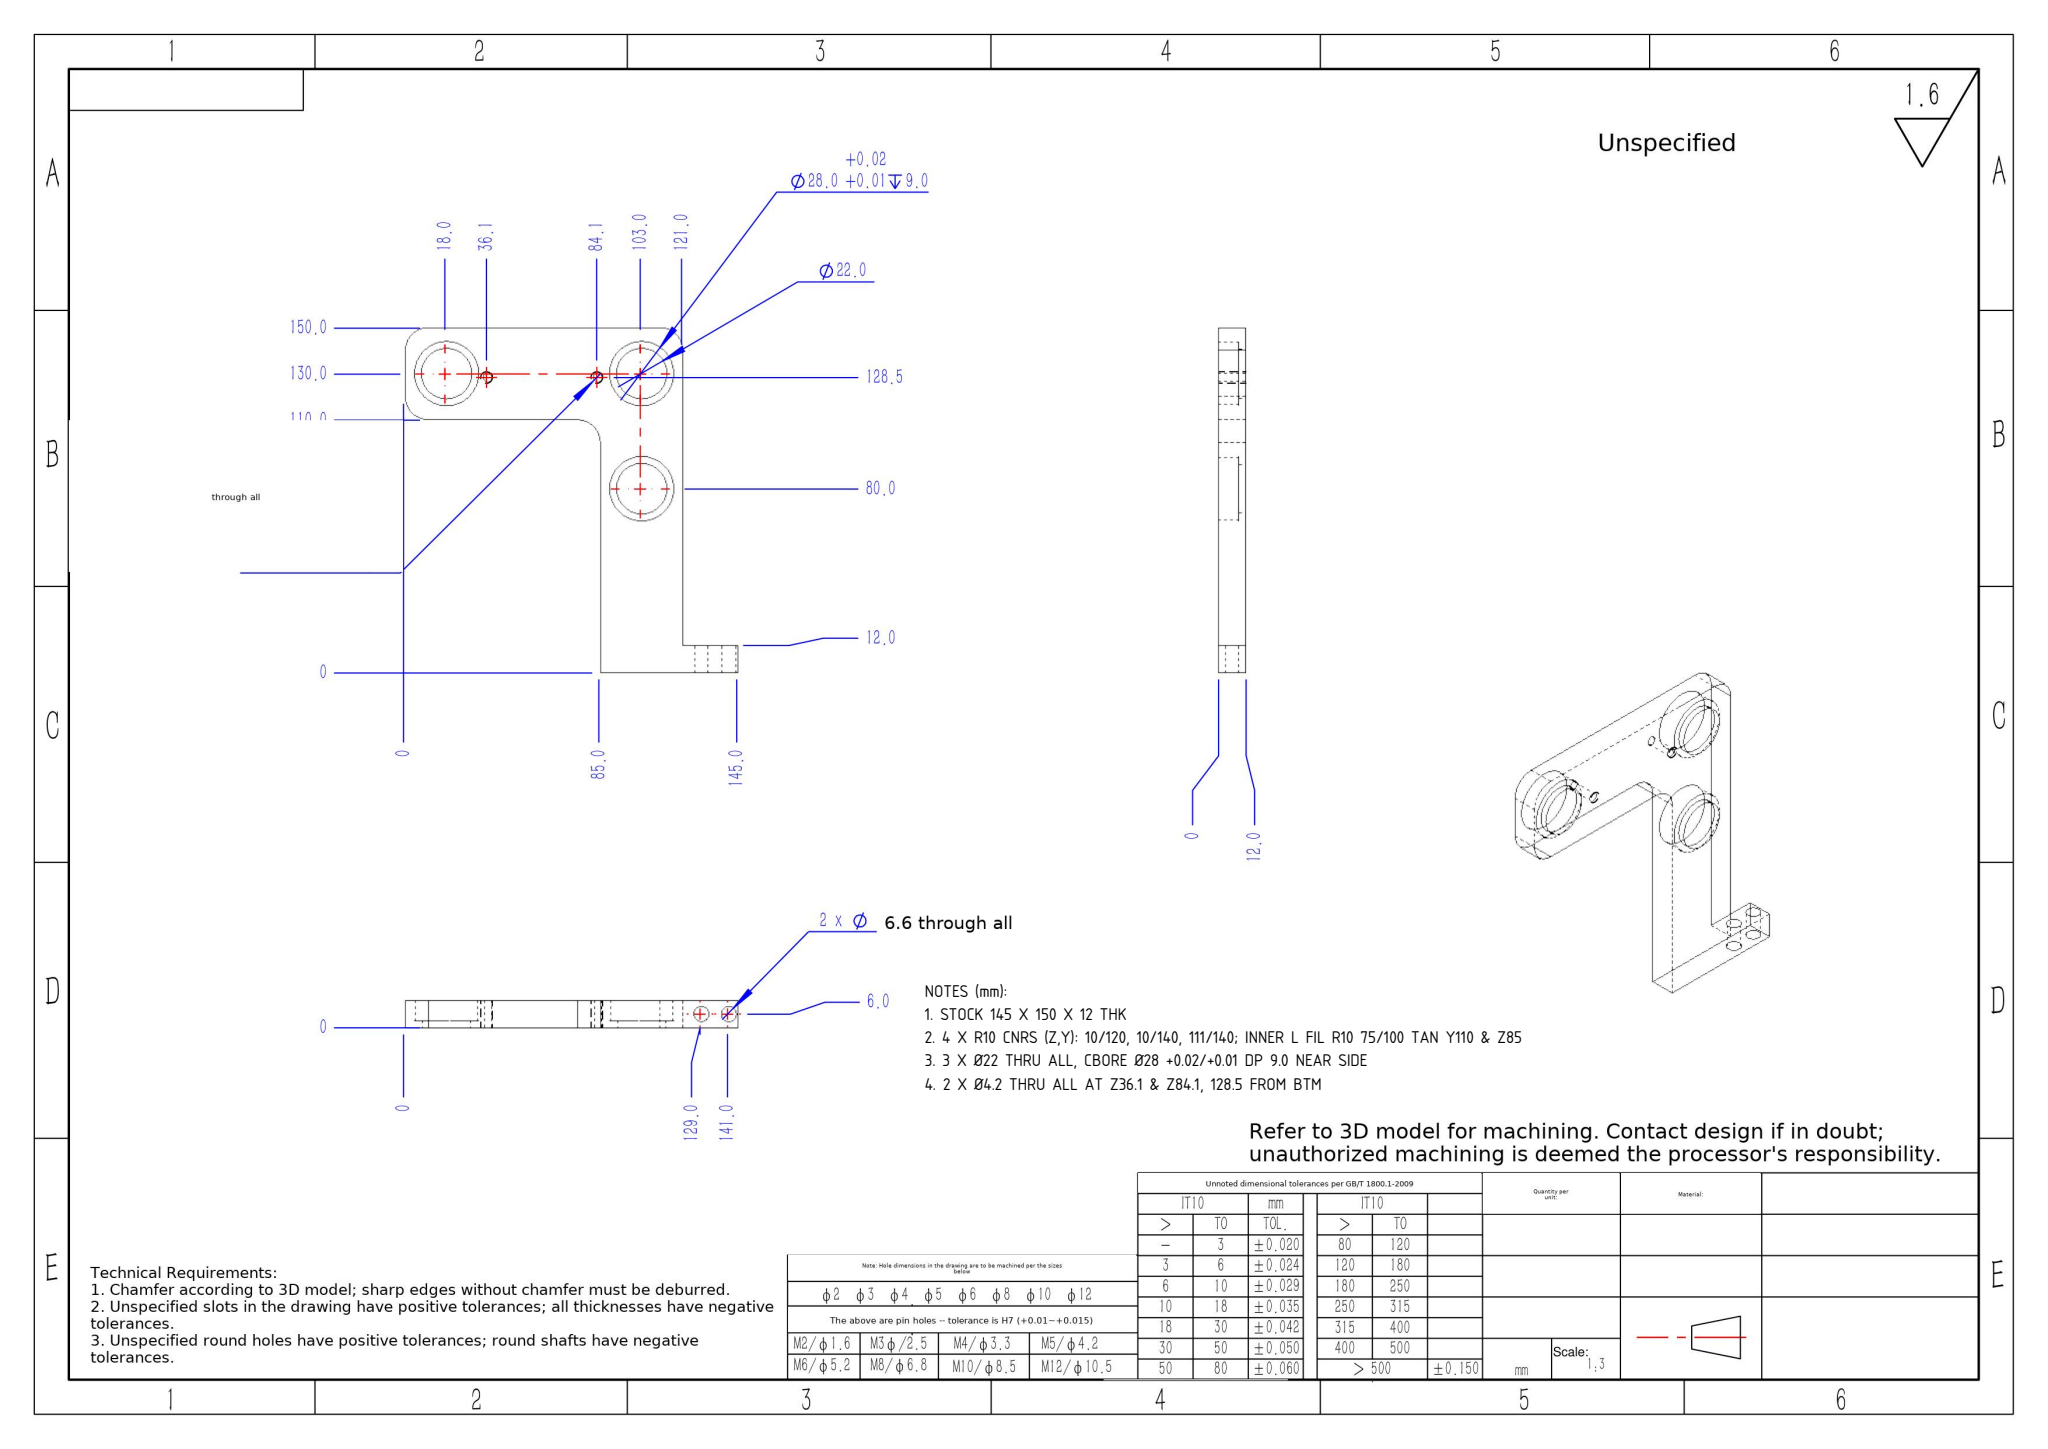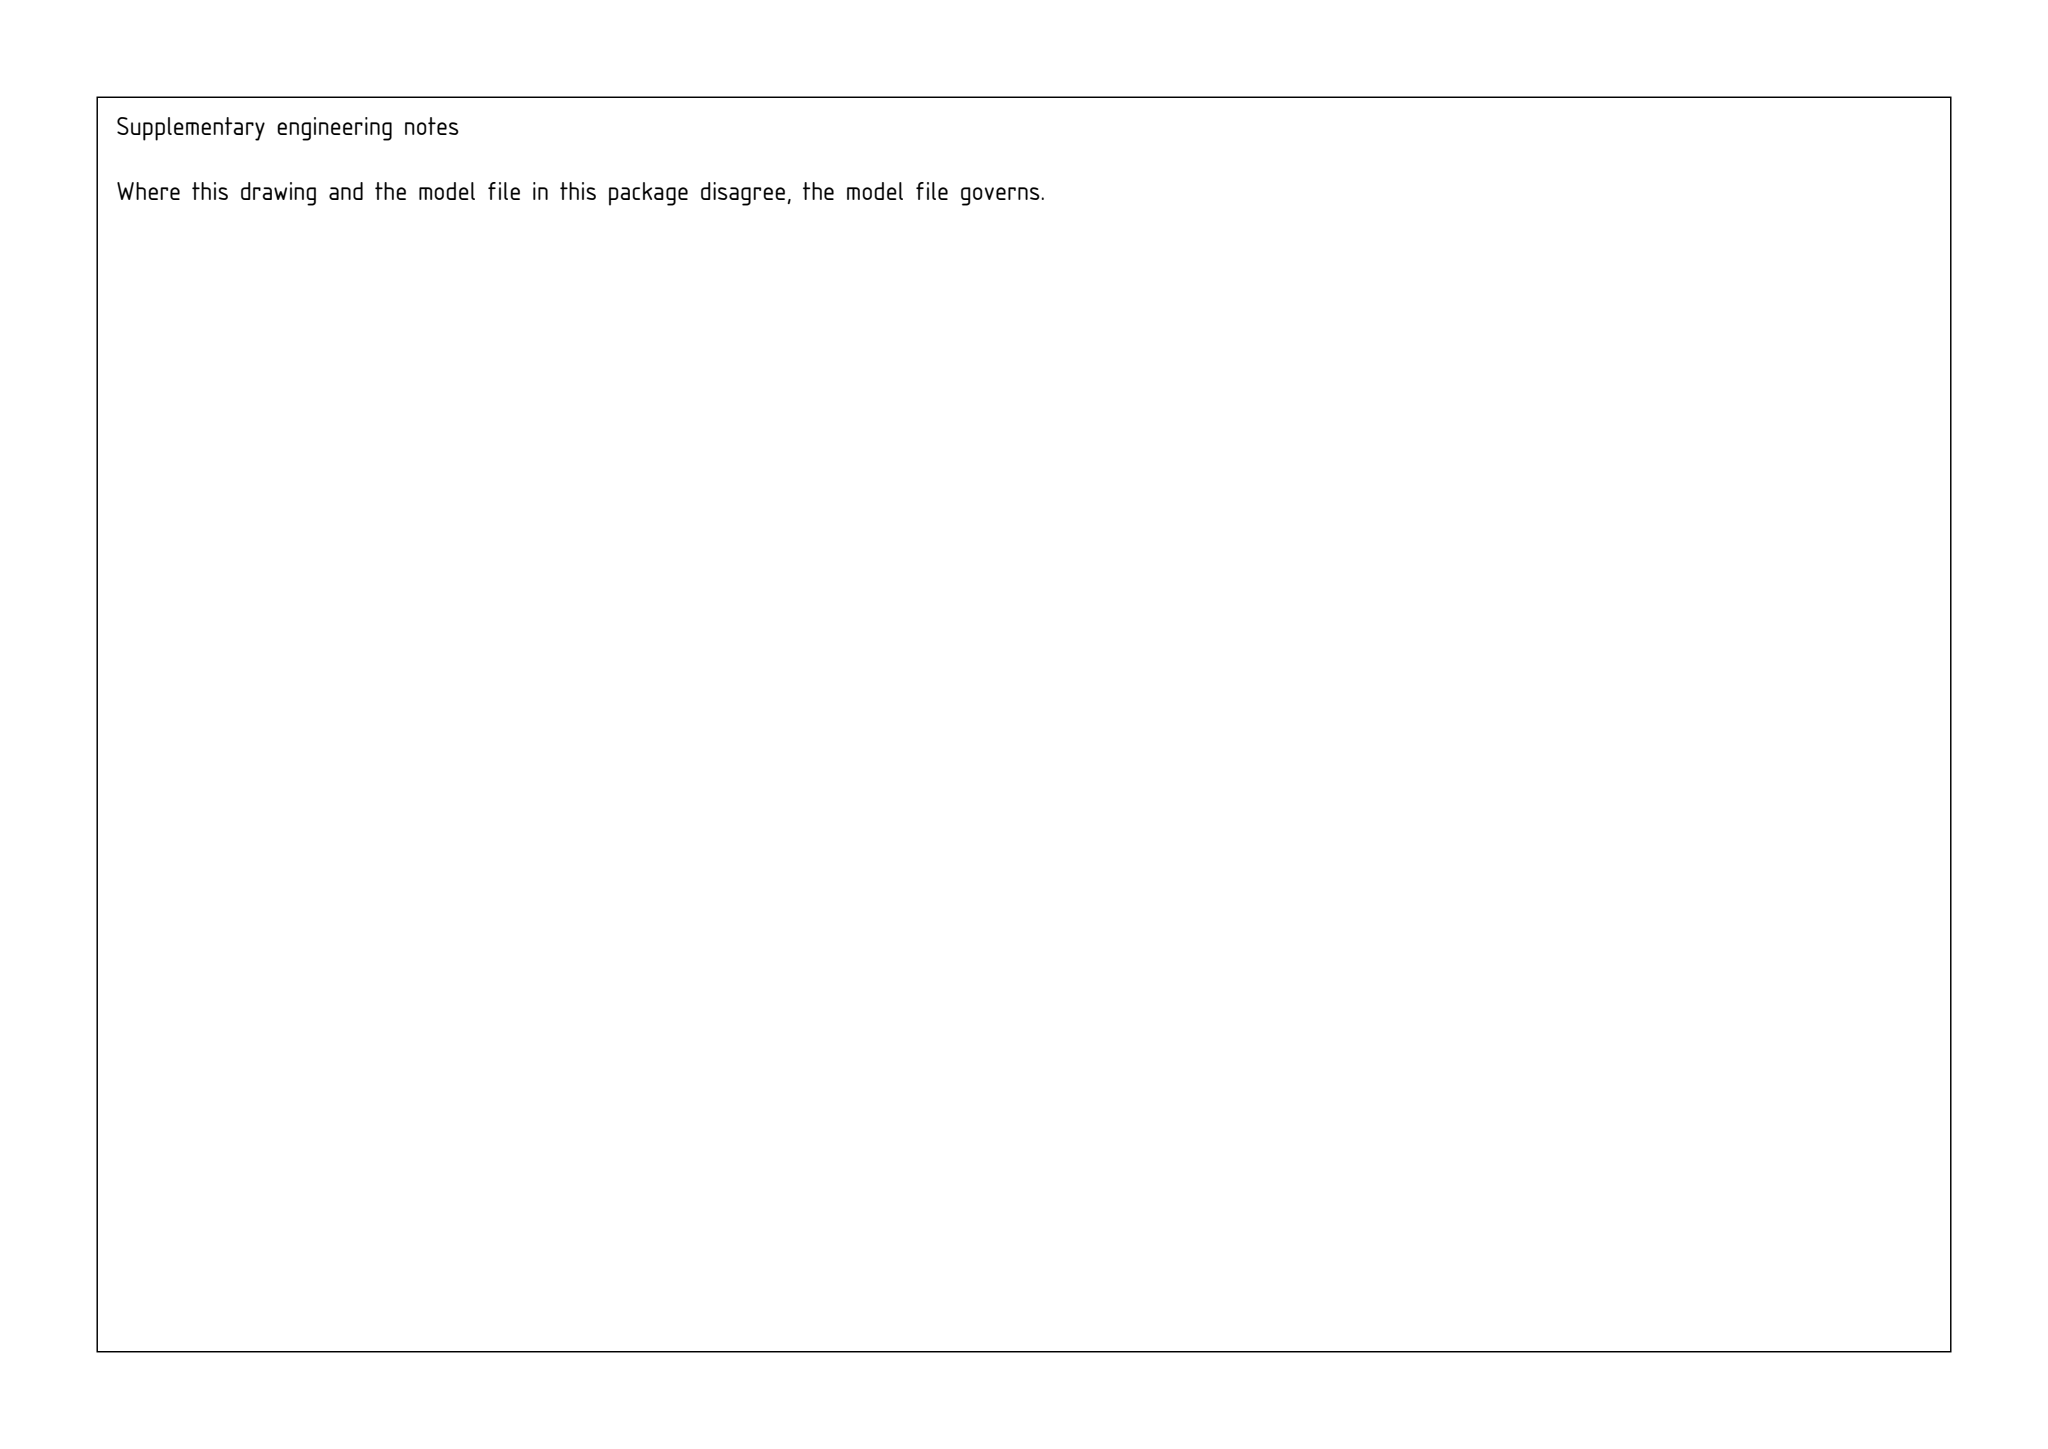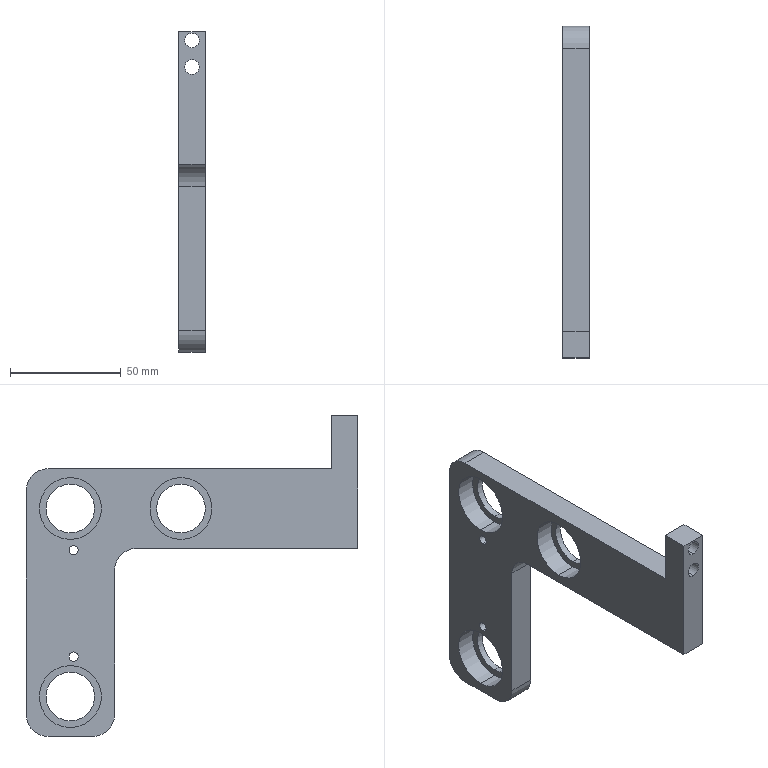Part | SolidWorks | mm | 1 solid | 37 faces | box 12 x 150 x 145 mm | volume 87341 mm3 | cylinder 24 | plane 13 | commonest cylinder face diameters 28 x6 22 x6 4.2 x4 6.6 x4 20 x4
Drawing notes:
STOCK 145 X 150 X 12 THK | from the solid: bbox_xyz [12.0,150.0,145.0]; z planes 0/145, y planes 0/150, x planes 0/12
4 X R10 CNRS (Z,Y): 10/120, 10/140, 111/140; INNER L FIL R10 75/100 TAN Y110 & Z85 | from the solid: Four Ø20 cyls axis x, len 12.0, at (y,z)=(120,10),(140,10),(140,111),(100,75); tangent planes y=110/150, z=0/85/121
3 X Ø22 THRU ALL, CBORE Ø28 +0.02/+0.01 DP 9.0 NEAR SIDE | from the solid: 3 x Ø28 L9.0 + Ø22 L3.0 coaxial at (y,z)=(130,18),(130,103),(80,103); 9+3=12 thk
2 X Ø4.2 THRU ALL AT Z36.1 & Z84.1, 128.5 FROM BTM | from the solid: cylinders Ø4.2, axis x, pos (y=128.5, z=36.11 & 84.11), length 12.0 = full thk
build123d program:
from build123d import *

# Parameters (mm, degrees)
SKETCH1_W            = 60
SKETCH1_H            = 150
BOSS_EXTRUDE1_DEPTH  = 12
SKETCH11_W           = 24
SKETCH11_H           = 138
CUT_EXTRUDE8_DEPTH   = 82.664
SKETCH12_R           = 11
CUT_EXTRUDE9_DEPTH   = 82.664
SKETCH13_R           = 14
CUT_EXTRUDE10_DEPTH  = 9
FILLET1_R            = 10
M6_CLEARANCE_HOLE1_D = 6.6
SKETCH19_W           = 12
SKETCH19_H           = 40
BOSS_EXTRUDE2_DEPTH  = 85
LPATTERN1_COUNT      = 2
LPATTERN1_PITCH      = 50
LPATTERN2_COUNT      = 2
LPATTERN2_PITCH      = 85
FILLET2_R            = 10
M5_TAPPED_HOLE1_D    = 4.2


with BuildPart() as part:
    # Sketch1 → Boss-Extrude1 (new body)
    with BuildSketch(Plane(origin=(0, 0, 0), x_dir=(0, 0, -1), z_dir=(1, 0, 0))):
        Rectangle(SKETCH1_W, SKETCH1_H)
    extrude(amount=BOSS_EXTRUDE1_DEPTH)

    # Sketch11 → Cut-Extrude8 (cut, through all)
    with BuildSketch(Plane(origin=(12, 0, 0), x_dir=(0, 0, -1), z_dir=(1, 0, 0))):
        with Locations((-18, 6)):
            Rectangle(SKETCH11_W, SKETCH11_H)
    extrude(amount=-CUT_EXTRUDE8_DEPTH, mode=Mode.SUBTRACT)

    # Sketch12 → Cut-Extrude9 (cut, through all)
    with BuildSketch(Plane(origin=(12, 0, 0), x_dir=(0, 0, -1), z_dir=(1, 0, 0))):
        with Locations((12, 55)):
            Circle(SKETCH12_R)
    cut_extrude9 = extrude(amount=-CUT_EXTRUDE9_DEPTH, mode=Mode.SUBTRACT)

    # Sketch13 → Cut-Extrude10 (cut)
    with BuildSketch(Plane.ZY):
        with Locations((-12, 55)):
            Circle(SKETCH13_R)
    cut_extrude10 = extrude(amount=-CUT_EXTRUDE10_DEPTH, mode=Mode.SUBTRACT)

    # Fillet1
    fillet1_edges = [part.edges().sort_by_distance(p)[0] for p in [
        (6, 75, 6),
    ]]
    fillet(fillet1_edges, radius=FILLET1_R)

    # M6 Clearance Hole1 (through all)
    with Locations(Plane(origin=(0, -63, 0), x_dir=(1, 0, 0), z_dir=(0, 1, 0))):
        with Locations((6, -14), (6, -26)):
            Hole(M6_CLEARANCE_HOLE1_D / 2)

    # Sketch19 → Boss-Extrude2 (add)
    with BuildSketch(Plane(origin=(0, 0, -30), x_dir=(-1, 0, 0), z_dir=(0, 0, -1))):
        with Locations((-6, 55)):
            Rectangle(SKETCH19_W, SKETCH19_H)
    extrude(amount=BOSS_EXTRUDE2_DEPTH)

    # LPattern1: Cut-Extrude9, Cut-Extrude10 ×2
    with Locations(*[(0, -i * LPATTERN1_PITCH, 0) for i in range(1, LPATTERN1_COUNT)]):
        add(cut_extrude9, mode=Mode.SUBTRACT)
        add(cut_extrude10, mode=Mode.SUBTRACT)

    # LPattern2: Cut-Extrude9, Cut-Extrude10 ×2
    with Locations(*[(0, 0, -i * LPATTERN2_PITCH) for i in range(1, LPATTERN2_COUNT)]):
        add(cut_extrude9, mode=Mode.SUBTRACT)
        add(cut_extrude10, mode=Mode.SUBTRACT)

    # Fillet2
    fillet2_edges = [part.edges().sort_by_distance(p)[0] for p in [
        (6, 35, -30),
        (6, 35, -115),
        (6, 75, -115),
    ]]
    fillet(fillet2_edges, radius=FILLET2_R)

    # M5 Tapped Hole1 (through all)
    with Locations(Plane(origin=(12, 0, 0), x_dir=(0, 0, -1), z_dir=(1, 0, 0))):
        with Locations((78.893, 53.5), (30.893, 53.5)):
            Hole(M5_TAPPED_HOLE1_D / 2)


solid = part.part